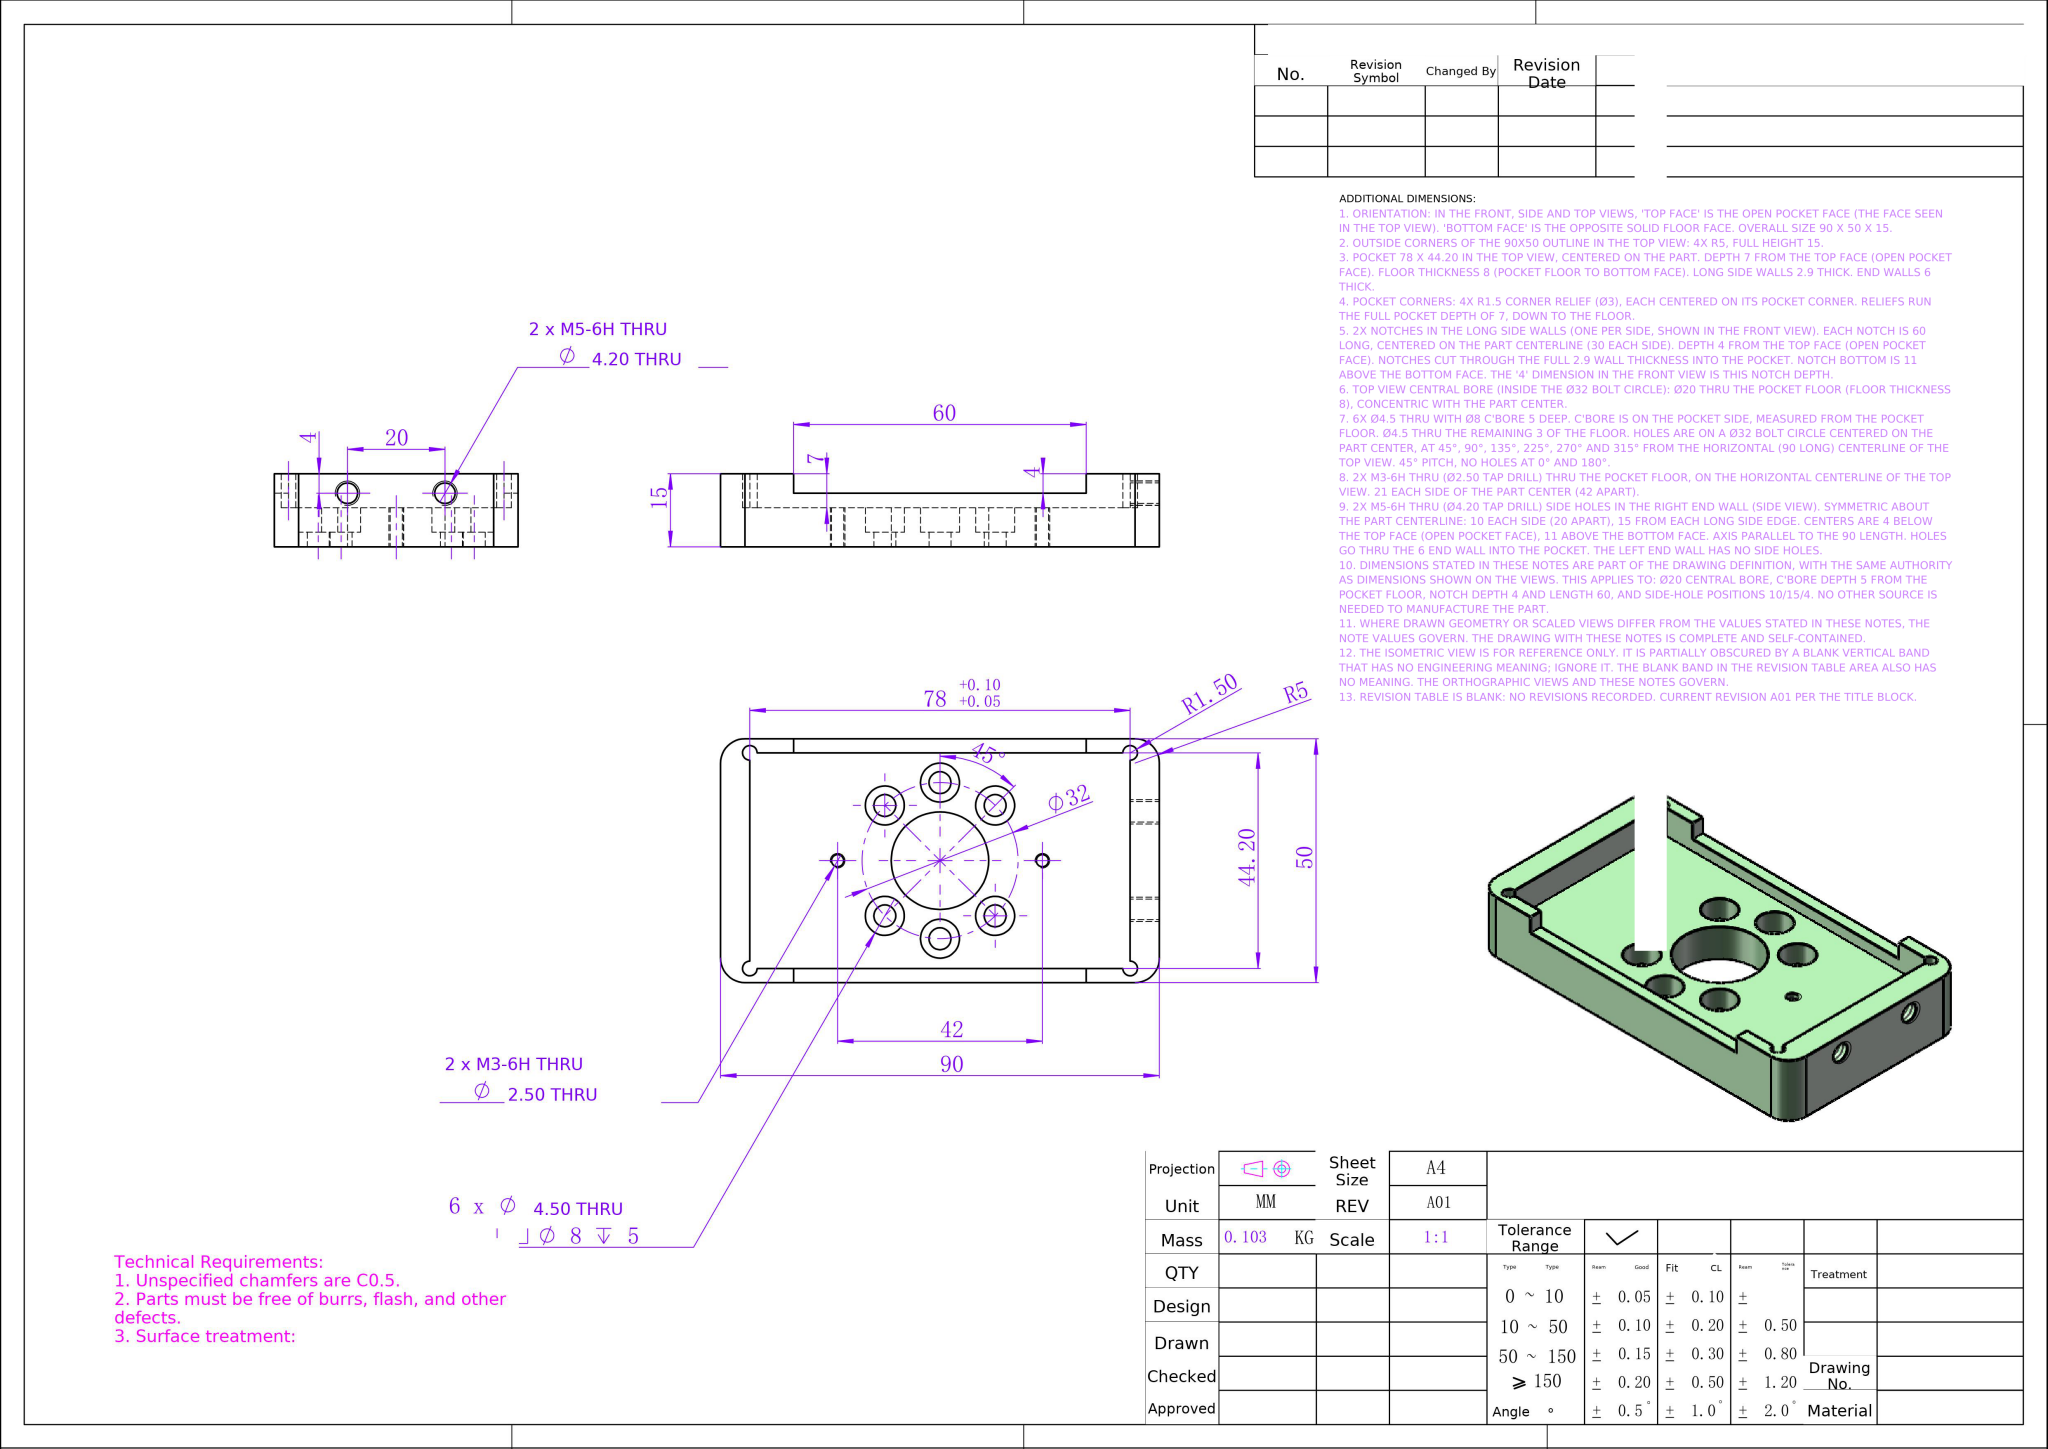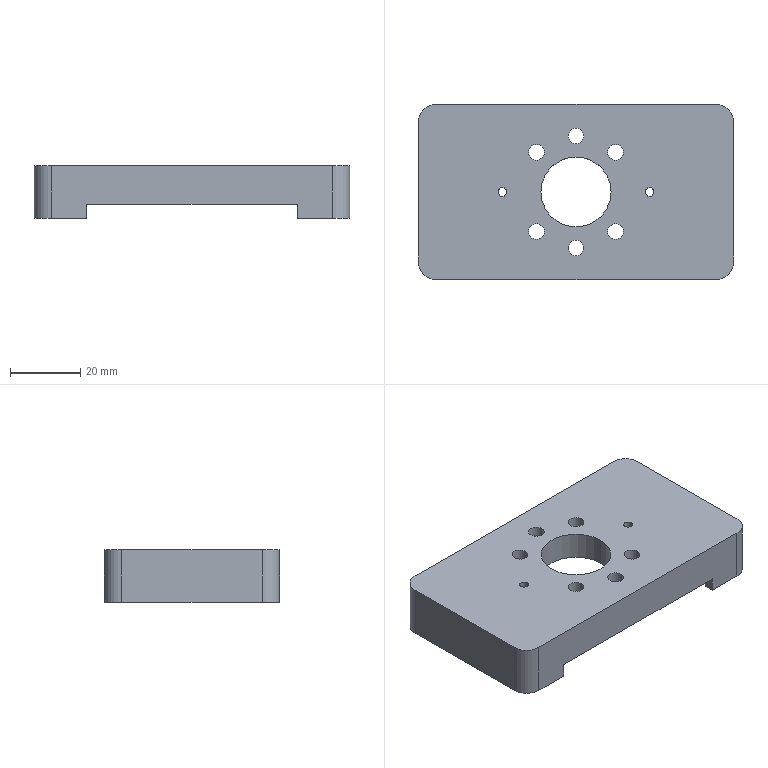Part | NX | mm | 1 solid | 68 faces | box 90 x 50 x 15 mm | volume 36952 mm3 | cylinder 44 | plane 24 | commonest cylinder face diameters 8 x12 4.5 x12 3 x6 4.2 x4 2.5 x4 10 x4 20 x2